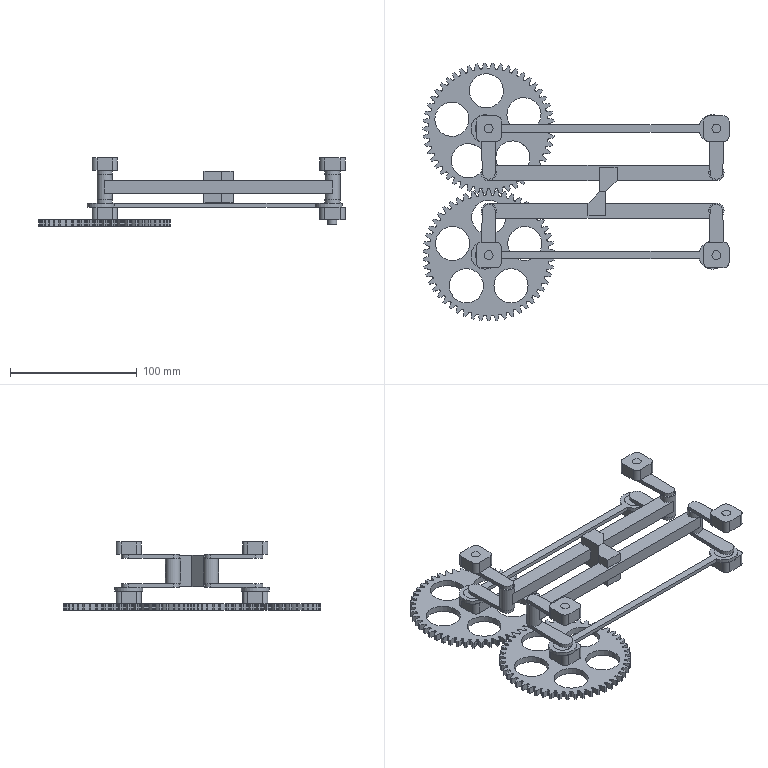Assembly | NX | mm | 24 component files | 24 solids | 860 faces | box 241.97 x 203.89 x 54 mm | volume 159802 mm3 | spline 500 | cylinder 204 | plane 156 | commonest cylinder face diameters 94.95 x100 8 x32 7 x18 12 x12 6 x12 27 x10 15 x8 10 x8
Bill of materials:
unnamed part 1 | 2 |  | Thin flat spur-gear-like disc with straight-extruded teeth all around the edge, five large round cutouts spaced evenly around the face, and a small round hole in the center.
unnamed part 2 | 1 |  | Crank-like lever: a flat arm with rounded ends that tapers along its length. A short cylindrical pin rises from the narrow end. At the wide end, a round disc sits below the arm, slightly off-center, and a longer cylindrical shaft extends downward from it.
unnamed part 3 | 1 |  | Crank-like lever: a flat tapered arm with rounded ends, a short upward pin at the narrow end, and a round disc plus a longer downward cylindrical shaft at the wide end.
unnamed part 4 | 2 |  | Very thin flat link: a long narrow straight strip joining two ring-shaped eyes, one at each end, each with a round through hole.
unnamed part 5 | 2 |  | Crank-like lever: a flat tapered arm with rounded ends, a short upward pin at the narrow end, and an offset round disc plus a longer downward cylindrical shaft at the wide end. Pin and shaft positions are swapped side-to-side compared with the similar lever parts.
unnamed part 6 | 8 |  | Square block with rounded vertical corners and a single round hole straight through the center from top to bottom.
unnamed part 7 | 2 |  | Long straight bar with a rectangular cross-section and a cylindrical boss at each end. Each boss has a small round through hole and is taller than the bar.
unnamed part 8 | 2 |  | Prismatic block whose top outline is a rectangle with one corner cut off at an angle, giving a five-sided shape. A rectangular slot is cut into one side face at mid-height.
unnamed part 9 | 4 |  | Crank-like lever: a flat tapered arm with rounded ends, a larger cylindrical pin rising from the wide end, and a smaller, shorter cylindrical pin extending downward from the narrow end.
Mates:
1. fix | gear 2 component
2. distance | gear 1 face | assembly datumplane
3. concentric | fix_block 8 edge | gear 2 edge
4. concentric | con_rod1 2 edge | fix_block 8 edge
5. concentric | con_rod2 2 edge | con_rod1 2 edge
6. concentric | con_rod5 4 arc | con_rod2 2 edge
7. concentric | fix_block 7 edge | con_rod5 4 edge
8. fix | assembly component
9. bond | fix_block 7 component | assembly component
10. bond | fix_block 8 component | assembly component
11. bond | con_rod1 2 component | assembly component
12. bond | con_rod5 4 component | assembly component
13. bond | fix_block 6 component | assembly component
14. bond | fix_block 5 component | assembly component
15. bond | con_rod1 1 component | assembly component
16. bond | con_rod5 3 component | assembly component
17. linear | assembly datumaxis | assembly cartesiancoordinatesystem | assembly cartesiancoordinatesystem
18. linear | assembly datumaxis | assembly cartesiancoordinatesystem | assembly cartesiancoordinatesystem
19. linear | assembly datumaxis | assembly cartesiancoordinatesystem | assembly cartesiancoordinatesystem
20. linear | assembly datumaxis | assembly cartesiancoordinatesystem | assembly cartesiancoordinatesystem
21. concentric | con_rod3 2 arc | con_rod1 2 edge
22. distance | gear 1 face | assembly datumplane